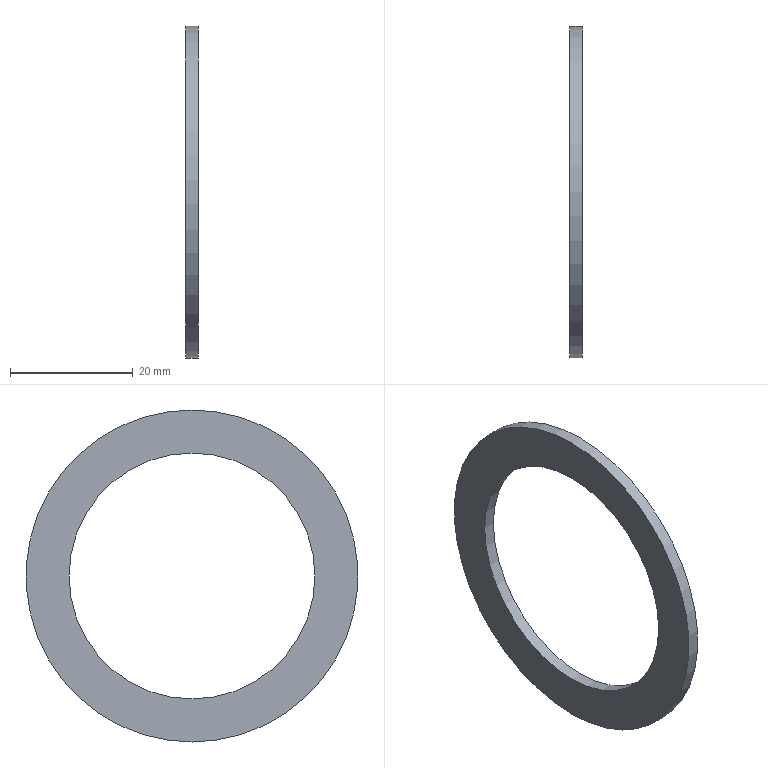Component | NX | LARGE_WASHER | 1 solid | 4 faces | box 2 x 54 x 54 mm | volume 2067 mm3 | cylinder 2 | plane 2 | commonest cylinder face diameters 54 x1 40 x1
STEP:
#1=CARTESIAN_POINT('',(0.,0.,0.));
#2=DIRECTION('',(0.,0.,1.));
#3=DIRECTION('',(1.,0.,0.));
#4=AXIS2_PLACEMENT_3D('',#1,#2,#3);
#5=CARTESIAN_POINT('',(-44.,-0.,26.));
#6=VERTEX_POINT('',#5);
#7=CARTESIAN_POINT('',(-44.,-0.,-1.));
#8=DIRECTION('',(-1.,0.,0.));
#9=DIRECTION('',(0.,0.,1.));
#10=AXIS2_PLACEMENT_3D('',#7,#8,#9);
#11=CIRCLE('',#10,27.);
#12=CARTESIAN_POINT('',(-44.,-0.,-1.));
#13=DIRECTION('',(1.,0.,0.));
#14=DIRECTION('',(0.,0.,-1.));
#15=AXIS2_PLACEMENT_3D('',#12,#13,#14);
#16=CYLINDRICAL_SURFACE('',#15,27.);
#17=CARTESIAN_POINT('',(9.425,0.));
#18=DIRECTION('',(-1.,0.));
#19=VECTOR('',#18,1.);
#20=LINE('',#17,#19);
#21=(GEOMETRIC_REPRESENTATION_CONTEXT(2)PARAMETRIC_REPRESENTATION_CONTEXT()REPRESENTATION_CONTEXT('',''));
#22=DEFINITIONAL_REPRESENTATION('',(#20),#21);
#23=PCURVE('',#16,#22);
#24=CARTESIAN_POINT('',(-44.,-0.,-1.));
#25=DIRECTION('',(-1.,0.,0.));
#26=DIRECTION('',(0.,0.,1.));
#27=AXIS2_PLACEMENT_3D('',#24,#25,#26);
#28=PLANE('',#27);
#29=CARTESIAN_POINT('',(0.,0.));
#30=DIRECTION('',(1.,0.));
#31=AXIS2_PLACEMENT_2D('',#29,#30);
#32=CIRCLE('',#31,27.);
#33=(GEOMETRIC_REPRESENTATION_CONTEXT(2)PARAMETRIC_REPRESENTATION_CONTEXT()REPRESENTATION_CONTEXT('',''));
#34=DEFINITIONAL_REPRESENTATION('',(#32),#33);
#35=PCURVE('',#28,#34);
#36=SURFACE_CURVE('',#11,(#23,#35),.PCURVE_S1.);
#37=EDGE_CURVE('',#6,#6,#36,.T.);
#38=ORIENTED_EDGE('',*,*,#37,.F.);
#39=CARTESIAN_POINT('',(-42.,-0.,26.));
#40=VERTEX_POINT('',#39);
#41=CARTESIAN_POINT('',(-44.,-0.,26.));
#42=CARTESIAN_POINT('',(-42.,-0.,26.));
#43=B_SPLINE_CURVE_WITH_KNOTS('',1,(#41,#42),.UNSPECIFIED.,.F.,.F.,(2,2),(0.,2.),.PIECEWISE_BEZIER_KNOTS.);
#44=CARTESIAN_POINT('',(9.425,0.));
#45=DIRECTION('',(0.,1.));
#46=VECTOR('',#45,1.);
#47=LINE('',#44,#46);
#48=(GEOMETRIC_REPRESENTATION_CONTEXT(2)PARAMETRIC_REPRESENTATION_CONTEXT()REPRESENTATION_CONTEXT('',''));
#49=DEFINITIONAL_REPRESENTATION('',(#47),#48);
#50=PCURVE('',#16,#49);
#51=CARTESIAN_POINT('',(3.142,0.));
#52=DIRECTION('',(0.,1.));
#53=VECTOR('',#52,1.);
#54=LINE('',#51,#53);
#55=(GEOMETRIC_REPRESENTATION_CONTEXT(2)PARAMETRIC_REPRESENTATION_CONTEXT()REPRESENTATION_CONTEXT('',''));
#56=DEFINITIONAL_REPRESENTATION('',(#54),#55);
#57=PCURVE('',#16,#56);
#58=SEAM_CURVE('',#43,(#50,#57),.PCURVE_S1.);
#59=EDGE_CURVE('',#6,#40,#58,.T.);
#60=ORIENTED_EDGE('',*,*,#59,.T.);
#61=CARTESIAN_POINT('',(-42.,-0.,-1.));
#62=DIRECTION('',(-1.,0.,0.));
#63=DIRECTION('',(0.,0.,1.));
#64=AXIS2_PLACEMENT_3D('',#61,#62,#63);
#65=CIRCLE('',#64,27.);
#66=CARTESIAN_POINT('',(9.425,2.));
#67=DIRECTION('',(-1.,0.));
#68=VECTOR('',#67,1.);
#69=LINE('',#66,#68);
#70=(GEOMETRIC_REPRESENTATION_CONTEXT(2)PARAMETRIC_REPRESENTATION_CONTEXT()REPRESENTATION_CONTEXT('',''));
#71=DEFINITIONAL_REPRESENTATION('',(#69),#70);
#72=PCURVE('',#16,#71);
#73=CARTESIAN_POINT('',(-42.,-0.,-1.));
#74=DIRECTION('',(-1.,0.,0.));
#75=DIRECTION('',(0.,0.,1.));
#76=AXIS2_PLACEMENT_3D('',#73,#74,#75);
#77=PLANE('',#76);
#78=CARTESIAN_POINT('',(0.,0.));
#79=DIRECTION('',(1.,0.));
#80=AXIS2_PLACEMENT_2D('',#78,#79);
#81=CIRCLE('',#80,27.);
#82=(GEOMETRIC_REPRESENTATION_CONTEXT(2)PARAMETRIC_REPRESENTATION_CONTEXT()REPRESENTATION_CONTEXT('',''));
#83=DEFINITIONAL_REPRESENTATION('',(#81),#82);
#84=PCURVE('',#77,#83);
#85=SURFACE_CURVE('',#65,(#72,#84),.PCURVE_S1.);
#86=EDGE_CURVE('',#40,#40,#85,.T.);
#87=ORIENTED_EDGE('',*,*,#86,.T.);
#88=ORIENTED_EDGE('',*,*,#59,.F.);
#89=EDGE_LOOP('',(#38,#60,#87,#88));
#90=FACE_BOUND('',#89,.T.);
#91=ADVANCED_FACE('',(#90),#16,.T.);
#92=CARTESIAN_POINT('',(-44.,-0.,19.));
#93=VERTEX_POINT('',#92);
#94=CARTESIAN_POINT('',(-44.,-0.,-1.));
#95=DIRECTION('',(-1.,0.,0.));
#96=DIRECTION('',(0.,0.,1.));
#97=AXIS2_PLACEMENT_3D('',#94,#95,#96);
#98=CIRCLE('',#97,20.);
#99=CARTESIAN_POINT('',(-44.,-0.,-1.));
#100=DIRECTION('',(1.,0.,0.));
#101=DIRECTION('',(0.,0.,-1.));
#102=AXIS2_PLACEMENT_3D('',#99,#100,#101);
#103=CYLINDRICAL_SURFACE('',#102,20.);
#104=CARTESIAN_POINT('',(9.425,0.));
#105=DIRECTION('',(-1.,0.));
#106=VECTOR('',#105,1.);
#107=LINE('',#104,#106);
#108=(GEOMETRIC_REPRESENTATION_CONTEXT(2)PARAMETRIC_REPRESENTATION_CONTEXT()REPRESENTATION_CONTEXT('',''));
#109=DEFINITIONAL_REPRESENTATION('',(#107),#108);
#110=PCURVE('',#103,#109);
#111=CARTESIAN_POINT('',(0.,0.));
#112=DIRECTION('',(1.,0.));
#113=AXIS2_PLACEMENT_2D('',#111,#112);
#114=CIRCLE('',#113,20.);
#115=(GEOMETRIC_REPRESENTATION_CONTEXT(2)PARAMETRIC_REPRESENTATION_CONTEXT()REPRESENTATION_CONTEXT('',''));
#116=DEFINITIONAL_REPRESENTATION('',(#114),#115);
#117=PCURVE('',#28,#116);
#118=SURFACE_CURVE('',#98,(#110,#117),.PCURVE_S1.);
#119=EDGE_CURVE('',#93,#93,#118,.T.);
#120=ORIENTED_EDGE('',*,*,#119,.F.);
#121=CARTESIAN_POINT('',(-42.,-0.,19.));
#122=VERTEX_POINT('',#121);
#123=CARTESIAN_POINT('',(-44.,-0.,19.));
#124=CARTESIAN_POINT('',(-42.,-0.,19.));
#125=B_SPLINE_CURVE_WITH_KNOTS('',1,(#123,#124),.UNSPECIFIED.,.F.,.F.,(2,2),(0.,2.),.PIECEWISE_BEZIER_KNOTS.);
#126=CARTESIAN_POINT('',(9.425,0.));
#127=DIRECTION('',(0.,1.));
#128=VECTOR('',#127,1.);
#129=LINE('',#126,#128);
#130=(GEOMETRIC_REPRESENTATION_CONTEXT(2)PARAMETRIC_REPRESENTATION_CONTEXT()REPRESENTATION_CONTEXT('',''));
#131=DEFINITIONAL_REPRESENTATION('',(#129),#130);
#132=PCURVE('',#103,#131);
#133=CARTESIAN_POINT('',(3.142,0.));
#134=DIRECTION('',(0.,1.));
#135=VECTOR('',#134,1.);
#136=LINE('',#133,#135);
#137=(GEOMETRIC_REPRESENTATION_CONTEXT(2)PARAMETRIC_REPRESENTATION_CONTEXT()REPRESENTATION_CONTEXT('',''));
#138=DEFINITIONAL_REPRESENTATION('',(#136),#137);
#139=PCURVE('',#103,#138);
#140=SEAM_CURVE('',#125,(#132,#139),.PCURVE_S1.);
#141=EDGE_CURVE('',#93,#122,#140,.T.);
#142=ORIENTED_EDGE('',*,*,#141,.T.);
#143=CARTESIAN_POINT('',(-42.,-0.,-1.));
#144=DIRECTION('',(-1.,0.,0.));
#145=DIRECTION('',(0.,0.,1.));
#146=AXIS2_PLACEMENT_3D('',#143,#144,#145);
#147=CIRCLE('',#146,20.);
#148=CARTESIAN_POINT('',(9.425,2.));
#149=DIRECTION('',(-1.,0.));
#150=VECTOR('',#149,1.);
#151=LINE('',#148,#150);
#152=(GEOMETRIC_REPRESENTATION_CONTEXT(2)PARAMETRIC_REPRESENTATION_CONTEXT()REPRESENTATION_CONTEXT('',''));
#153=DEFINITIONAL_REPRESENTATION('',(#151),#152);
#154=PCURVE('',#103,#153);
#155=CARTESIAN_POINT('',(0.,0.));
#156=DIRECTION('',(1.,0.));
#157=AXIS2_PLACEMENT_2D('',#155,#156);
#158=CIRCLE('',#157,20.);
#159=(GEOMETRIC_REPRESENTATION_CONTEXT(2)PARAMETRIC_REPRESENTATION_CONTEXT()REPRESENTATION_CONTEXT('',''));
#160=DEFINITIONAL_REPRESENTATION('',(#158),#159);
#161=PCURVE('',#77,#160);
#162=SURFACE_CURVE('',#147,(#154,#161),.PCURVE_S1.);
#163=EDGE_CURVE('',#122,#122,#162,.T.);
#164=ORIENTED_EDGE('',*,*,#163,.T.);
#165=ORIENTED_EDGE('',*,*,#141,.F.);
#166=EDGE_LOOP('',(#120,#142,#164,#165));
#167=FACE_BOUND('',#166,.F.);
#168=ADVANCED_FACE('',(#167),#103,.F.);
#169=ORIENTED_EDGE('',*,*,#37,.T.);
#170=EDGE_LOOP('',(#169));
#171=FACE_BOUND('',#170,.T.);
#172=ORIENTED_EDGE('',*,*,#119,.F.);
#173=EDGE_LOOP('',(#172));
#174=FACE_BOUND('',#173,.T.);
#175=ADVANCED_FACE('',(#171,#174),#28,.T.);
#176=ORIENTED_EDGE('',*,*,#86,.F.);
#177=EDGE_LOOP('',(#176));
#178=FACE_BOUND('',#177,.T.);
#179=ORIENTED_EDGE('',*,*,#163,.T.);
#180=EDGE_LOOP('',(#179));
#181=FACE_BOUND('',#180,.T.);
#182=ADVANCED_FACE('',(#178,#181),#77,.F.);
#183=CLOSED_SHELL('',(#91,#168,#175,#182));
#184=MANIFOLD_SOLID_BREP('',#183);
#185=(LENGTH_UNIT()NAMED_UNIT(*)SI_UNIT(.MILLI.,.METRE.));
#186=UNCERTAINTY_MEASURE_WITH_UNIT(LENGTH_MEASURE(0.00001),#185,'','');
#187=(NAMED_UNIT(*)PLANE_ANGLE_UNIT()SI_UNIT($,.RADIAN.));
#188=(NAMED_UNIT(*)SI_UNIT($,.STERADIAN.)SOLID_ANGLE_UNIT());
#189=(GEOMETRIC_REPRESENTATION_CONTEXT(3)GLOBAL_UNCERTAINTY_ASSIGNED_CONTEXT((#186))GLOBAL_UNIT_ASSIGNED_CONTEXT((#185,#187,#188))REPRESENTATION_CONTEXT('',''));
#190=ADVANCED_BREP_SHAPE_REPRESENTATION('',(#4,#184),#189);